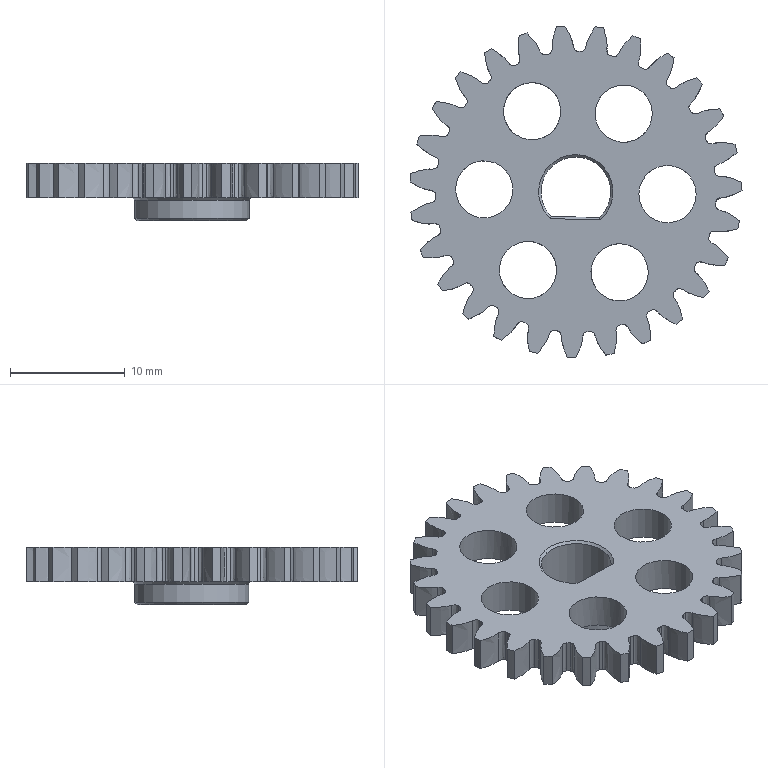Component | NX | DJZ_03_GEAR2 | 1 solid | 178 faces | volume 1367 mm3 | other 135 | cylinder 35 | plane 5 | cone 3 | commonest cylinder face diameters 24.5 x27 5 x6 10 x1 6.1 x1